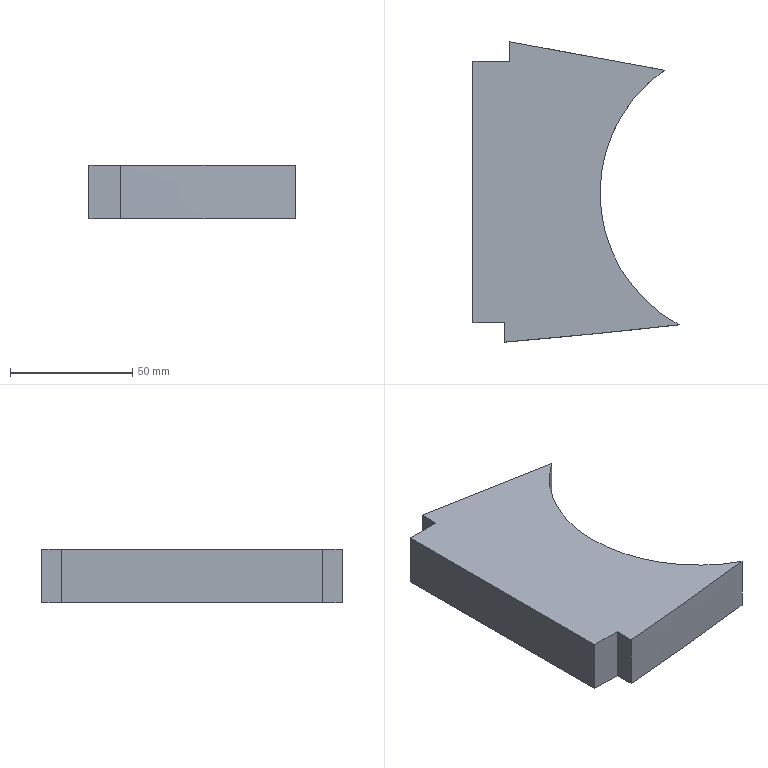Component | NX | AILERON_RIB_2 | 1 solid | 19 faces | volume 29944 mm3 | plane 13 | other 2 | cylinder 2 | spline 2 | commonest cylinder face diameters 122.237 x1 126.237 x1